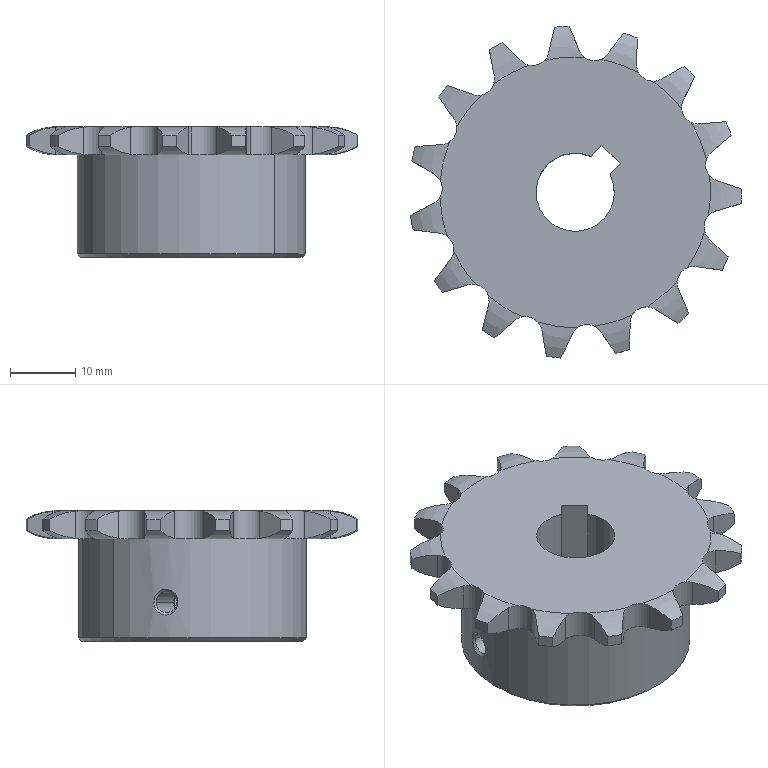Component | SolidWorks | LD101-02-35B15-d12-1 | 1 solid | 118 faces | volume 19259 mm3 | cylinder 44 | plane 36 | spline 32 | cone 6 | commonest cylinder face diameters 5.08 x20 51 x15 3.242 x4 12 x3 35 x2